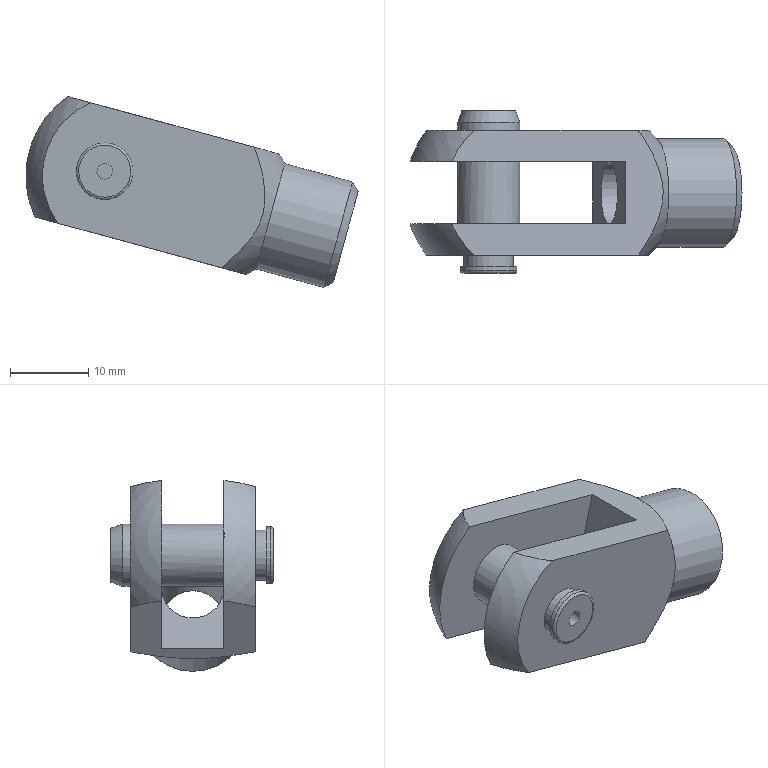Component | NX | F-MA20Y | 1 solid | 28 faces | volume 5790 mm3 | plane 15 | cylinder 7 | cone 3 | sphere 2 | torus 1 | commonest cylinder face diameters 8 x3 14 x1 2 x1 7.273 x1 6.4 x1